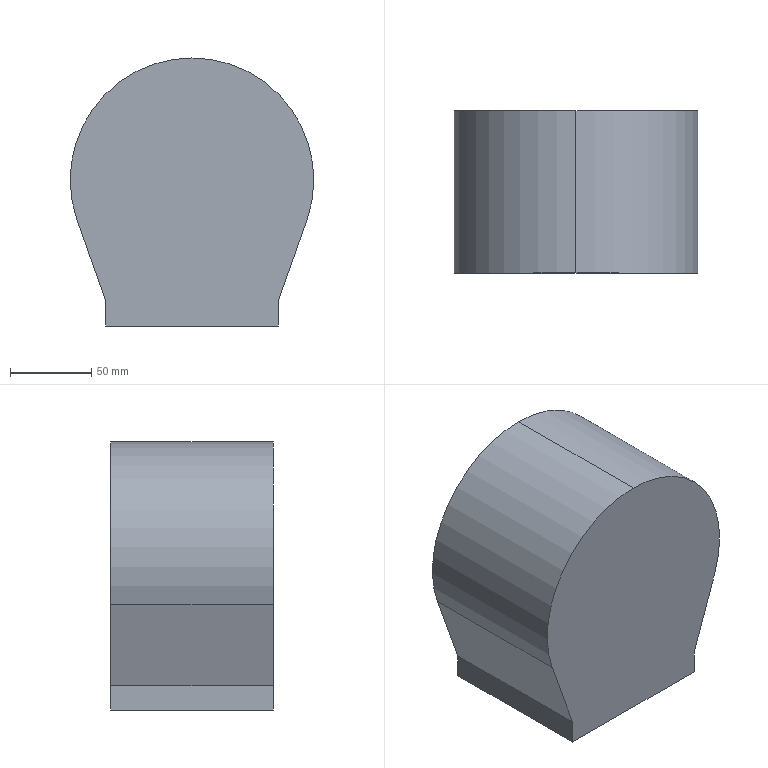Component | SolidWorks | ArmHousing-1 | 1 solid | 33 faces | box 150 x 100 x 165 mm | volume 519857 mm3 | plane 21 | cylinder 12 | commonest cylinder face diameters 4 x8 146 x2 150 x2
STEP:
#1=COLOUR_RGB('',0.7922,0.8196,0.9333);
#2=FILL_AREA_STYLE_COLOUR('',#1);
#3=FILL_AREA_STYLE('',(#2));
#4=SURFACE_STYLE_FILL_AREA(#3);
#5=SURFACE_SIDE_STYLE('',(#4));
#6=SURFACE_STYLE_USAGE(.BOTH.,#5);
#7=PRESENTATION_STYLE_ASSIGNMENT((#6));
#8=CARTESIAN_POINT('',(21.418,34.134,-80.807));
#9=VERTEX_POINT('',#8);
#10=CARTESIAN_POINT('',(21.418,34.134,-80.65));
#11=VERTEX_POINT('',#10);
#12=CARTESIAN_POINT('',(21.418,34.134,-80.729));
#13=DIRECTION('',(0.,1.,-0.));
#14=DIRECTION('',(0.,0.,1.));
#15=AXIS2_PLACEMENT_3D('',#12,#13,#14);
#16=CIRCLE('',#15,0.07874);
#17=EDGE_CURVE('',#9,#11,#16,.T.);
#18=ORIENTED_EDGE('',*,*,#17,.F.);
#19=CARTESIAN_POINT('',(21.418,34.724,-80.807));
#20=VERTEX_POINT('',#19);
#21=CARTESIAN_POINT('',(21.418,34.134,-80.807));
#22=DIRECTION('',(0.,1.,-0.));
#23=VECTOR('',#22,39.37);
#24=LINE('',#21,#23);
#25=EDGE_CURVE('',#9,#20,#24,.T.);
#26=ORIENTED_EDGE('',*,*,#25,.T.);
#27=CARTESIAN_POINT('',(21.418,34.724,-80.65));
#28=VERTEX_POINT('',#27);
#29=CARTESIAN_POINT('',(21.418,34.724,-80.729));
#30=DIRECTION('',(0.,1.,-0.));
#31=DIRECTION('',(0.,0.,1.));
#32=AXIS2_PLACEMENT_3D('',#29,#30,#31);
#33=CIRCLE('',#32,0.07874);
#34=EDGE_CURVE('',#20,#28,#33,.T.);
#35=ORIENTED_EDGE('',*,*,#34,.T.);
#36=CARTESIAN_POINT('',(21.418,34.134,-80.65));
#37=DIRECTION('',(0.,1.,-0.));
#38=VECTOR('',#37,39.37);
#39=LINE('',#36,#38);
#40=EDGE_CURVE('',#11,#28,#39,.T.);
#41=ORIENTED_EDGE('',*,*,#40,.F.);
#42=EDGE_LOOP('',(#18,#26,#35,#41));
#43=FACE_OUTER_BOUND('',#42,.T.);
#44=CARTESIAN_POINT('',(21.418,34.134,-80.729));
#45=DIRECTION('',(0.,1.,-0.));
#46=DIRECTION('',(0.,0.,1.));
#47=AXIS2_PLACEMENT_3D('',#44,#45,#46);
#48=CYLINDRICAL_SURFACE('',#47,0.07874);
#49=ADVANCED_FACE('',(#43),#48,.F.);
#50=CARTESIAN_POINT('',(24.758,34.134,-80.807));
#51=VERTEX_POINT('',#50);
#52=CARTESIAN_POINT('',(24.758,34.134,-80.65));
#53=VERTEX_POINT('',#52);
#54=CARTESIAN_POINT('',(24.758,34.134,-80.729));
#55=DIRECTION('',(0.,1.,-0.));
#56=DIRECTION('',(0.,0.,1.));
#57=AXIS2_PLACEMENT_3D('',#54,#55,#56);
#58=CIRCLE('',#57,0.07874);
#59=EDGE_CURVE('',#51,#53,#58,.T.);
#60=ORIENTED_EDGE('',*,*,#59,.F.);
#61=CARTESIAN_POINT('',(24.758,34.724,-80.807));
#62=VERTEX_POINT('',#61);
#63=CARTESIAN_POINT('',(24.758,34.134,-80.807));
#64=DIRECTION('',(0.,1.,-0.));
#65=VECTOR('',#64,39.37);
#66=LINE('',#63,#65);
#67=EDGE_CURVE('',#51,#62,#66,.T.);
#68=ORIENTED_EDGE('',*,*,#67,.T.);
#69=CARTESIAN_POINT('',(24.758,34.724,-80.65));
#70=VERTEX_POINT('',#69);
#71=CARTESIAN_POINT('',(24.758,34.724,-80.729));
#72=DIRECTION('',(0.,1.,-0.));
#73=DIRECTION('',(0.,0.,1.));
#74=AXIS2_PLACEMENT_3D('',#71,#72,#73);
#75=CIRCLE('',#74,0.07874);
#76=EDGE_CURVE('',#62,#70,#75,.T.);
#77=ORIENTED_EDGE('',*,*,#76,.T.);
#78=CARTESIAN_POINT('',(24.758,34.134,-80.65));
#79=DIRECTION('',(0.,1.,-0.));
#80=VECTOR('',#79,39.37);
#81=LINE('',#78,#80);
#82=EDGE_CURVE('',#53,#70,#81,.T.);
#83=ORIENTED_EDGE('',*,*,#82,.F.);
#84=EDGE_LOOP('',(#60,#68,#77,#83));
#85=FACE_OUTER_BOUND('',#84,.T.);
#86=CARTESIAN_POINT('',(24.758,34.134,-80.729));
#87=DIRECTION('',(0.,1.,-0.));
#88=DIRECTION('',(0.,0.,1.));
#89=AXIS2_PLACEMENT_3D('',#86,#87,#88);
#90=CYLINDRICAL_SURFACE('',#89,0.07874);
#91=ADVANCED_FACE('',(#85),#90,.F.);
#92=CARTESIAN_POINT('',(24.758,34.134,-84.148));
#93=VERTEX_POINT('',#92);
#94=CARTESIAN_POINT('',(24.758,34.134,-83.991));
#95=VERTEX_POINT('',#94);
#96=CARTESIAN_POINT('',(24.758,34.134,-84.069));
#97=DIRECTION('',(0.,1.,-0.));
#98=DIRECTION('',(0.,0.,1.));
#99=AXIS2_PLACEMENT_3D('',#96,#97,#98);
#100=CIRCLE('',#99,0.07874);
#101=EDGE_CURVE('',#93,#95,#100,.T.);
#102=ORIENTED_EDGE('',*,*,#101,.F.);
#103=CARTESIAN_POINT('',(24.758,34.724,-84.148));
#104=VERTEX_POINT('',#103);
#105=CARTESIAN_POINT('',(24.758,34.134,-84.148));
#106=DIRECTION('',(0.,1.,-0.));
#107=VECTOR('',#106,39.37);
#108=LINE('',#105,#107);
#109=EDGE_CURVE('',#93,#104,#108,.T.);
#110=ORIENTED_EDGE('',*,*,#109,.T.);
#111=CARTESIAN_POINT('',(24.758,34.724,-83.991));
#112=VERTEX_POINT('',#111);
#113=CARTESIAN_POINT('',(24.758,34.724,-84.069));
#114=DIRECTION('',(0.,1.,-0.));
#115=DIRECTION('',(0.,0.,1.));
#116=AXIS2_PLACEMENT_3D('',#113,#114,#115);
#117=CIRCLE('',#116,0.07874);
#118=EDGE_CURVE('',#104,#112,#117,.T.);
#119=ORIENTED_EDGE('',*,*,#118,.T.);
#120=CARTESIAN_POINT('',(24.758,34.134,-83.991));
#121=DIRECTION('',(0.,1.,-0.));
#122=VECTOR('',#121,39.37);
#123=LINE('',#120,#122);
#124=EDGE_CURVE('',#95,#112,#123,.T.);
#125=ORIENTED_EDGE('',*,*,#124,.F.);
#126=EDGE_LOOP('',(#102,#110,#119,#125));
#127=FACE_OUTER_BOUND('',#126,.T.);
#128=CARTESIAN_POINT('',(24.758,34.134,-84.069));
#129=DIRECTION('',(0.,1.,-0.));
#130=DIRECTION('',(0.,0.,1.));
#131=AXIS2_PLACEMENT_3D('',#128,#129,#130);
#132=CYLINDRICAL_SURFACE('',#131,0.07874);
#133=ADVANCED_FACE('',(#127),#132,.F.);
#134=CARTESIAN_POINT('',(21.418,34.134,-84.148));
#135=VERTEX_POINT('',#134);
#136=CARTESIAN_POINT('',(21.418,34.134,-83.991));
#137=VERTEX_POINT('',#136);
#138=CARTESIAN_POINT('',(21.418,34.134,-84.069));
#139=DIRECTION('',(0.,1.,-0.));
#140=DIRECTION('',(0.,0.,1.));
#141=AXIS2_PLACEMENT_3D('',#138,#139,#140);
#142=CIRCLE('',#141,0.07874);
#143=EDGE_CURVE('',#135,#137,#142,.T.);
#144=ORIENTED_EDGE('',*,*,#143,.F.);
#145=CARTESIAN_POINT('',(21.418,34.724,-84.148));
#146=VERTEX_POINT('',#145);
#147=CARTESIAN_POINT('',(21.418,34.134,-84.148));
#148=DIRECTION('',(0.,1.,-0.));
#149=VECTOR('',#148,39.37);
#150=LINE('',#147,#149);
#151=EDGE_CURVE('',#135,#146,#150,.T.);
#152=ORIENTED_EDGE('',*,*,#151,.T.);
#153=CARTESIAN_POINT('',(21.418,34.724,-83.991));
#154=VERTEX_POINT('',#153);
#155=CARTESIAN_POINT('',(21.418,34.724,-84.069));
#156=DIRECTION('',(0.,1.,-0.));
#157=DIRECTION('',(0.,0.,1.));
#158=AXIS2_PLACEMENT_3D('',#155,#156,#157);
#159=CIRCLE('',#158,0.07874);
#160=EDGE_CURVE('',#146,#154,#159,.T.);
#161=ORIENTED_EDGE('',*,*,#160,.T.);
#162=CARTESIAN_POINT('',(21.418,34.134,-83.991));
#163=DIRECTION('',(0.,1.,-0.));
#164=VECTOR('',#163,39.37);
#165=LINE('',#162,#164);
#166=EDGE_CURVE('',#137,#154,#165,.T.);
#167=ORIENTED_EDGE('',*,*,#166,.F.);
#168=EDGE_LOOP('',(#144,#152,#161,#167));
#169=FACE_OUTER_BOUND('',#168,.T.);
#170=CARTESIAN_POINT('',(21.418,34.134,-84.069));
#171=DIRECTION('',(0.,1.,-0.));
#172=DIRECTION('',(0.,0.,1.));
#173=AXIS2_PLACEMENT_3D('',#170,#171,#172);
#174=CYLINDRICAL_SURFACE('',#173,0.07874);
#175=ADVANCED_FACE('',(#169),#174,.F.);
#176=CARTESIAN_POINT('',(23.088,34.724,-79.525));
#177=VERTEX_POINT('',#176);
#178=CARTESIAN_POINT('',(25.796,34.724,-83.361));
#179=VERTEX_POINT('',#178);
#180=CARTESIAN_POINT('',(23.088,34.724,-82.399));
#181=DIRECTION('',(0.,1.,-0.));
#182=DIRECTION('',(0.,0.,1.));
#183=AXIS2_PLACEMENT_3D('',#180,#181,#182);
#184=CIRCLE('',#183,2.874);
#185=EDGE_CURVE('',#177,#179,#184,.T.);
#186=ORIENTED_EDGE('',*,*,#185,.F.);
#187=CARTESIAN_POINT('',(23.088,37.795,-79.525));
#188=VERTEX_POINT('',#187);
#189=CARTESIAN_POINT('',(23.088,25.507,-79.525));
#190=DIRECTION('',(0.,1.,-0.));
#191=VECTOR('',#190,39.37);
#192=LINE('',#189,#191);
#193=EDGE_CURVE('',#177,#188,#192,.T.);
#194=ORIENTED_EDGE('',*,*,#193,.T.);
#195=CARTESIAN_POINT('',(25.796,37.795,-83.361));
#196=VERTEX_POINT('',#195);
#197=CARTESIAN_POINT('',(23.088,37.795,-82.399));
#198=DIRECTION('',(0.,1.,-0.));
#199=DIRECTION('',(0.,0.,1.));
#200=AXIS2_PLACEMENT_3D('',#197,#198,#199);
#201=CIRCLE('',#200,2.874);
#202=EDGE_CURVE('',#188,#196,#201,.T.);
#203=ORIENTED_EDGE('',*,*,#202,.T.);
#204=CARTESIAN_POINT('',(25.796,25.507,-83.361));
#205=DIRECTION('',(0.,1.,-0.));
#206=VECTOR('',#205,39.37);
#207=LINE('',#204,#206);
#208=EDGE_CURVE('',#179,#196,#207,.T.);
#209=ORIENTED_EDGE('',*,*,#208,.F.);
#210=EDGE_LOOP('',(#186,#194,#203,#209));
#211=FACE_OUTER_BOUND('',#210,.T.);
#212=CARTESIAN_POINT('',(23.088,25.507,-82.399));
#213=DIRECTION('',(0.,1.,-0.));
#214=DIRECTION('',(0.,0.,1.));
#215=AXIS2_PLACEMENT_3D('',#212,#213,#214);
#216=CYLINDRICAL_SURFACE('',#215,2.874);
#217=ADVANCED_FACE('',(#211),#216,.F.);
#218=CARTESIAN_POINT('',(20.306,33.858,-83.387));
#219=VERTEX_POINT('',#218);
#220=CARTESIAN_POINT('',(23.088,33.858,-79.446));
#221=VERTEX_POINT('',#220);
#222=CARTESIAN_POINT('',(23.088,33.858,-82.399));
#223=DIRECTION('',(0.,1.,-0.));
#224=DIRECTION('',(0.,0.,-1.));
#225=AXIS2_PLACEMENT_3D('',#222,#223,#224);
#226=CIRCLE('',#225,2.953);
#227=EDGE_CURVE('',#219,#221,#226,.T.);
#228=ORIENTED_EDGE('',*,*,#227,.T.);
#229=CARTESIAN_POINT('',(23.088,37.795,-79.446));
#230=VERTEX_POINT('',#229);
#231=CARTESIAN_POINT('',(23.088,25.507,-79.446));
#232=DIRECTION('',(0.,1.,-0.));
#233=VECTOR('',#232,39.37);
#234=LINE('',#231,#233);
#235=EDGE_CURVE('',#221,#230,#234,.T.);
#236=ORIENTED_EDGE('',*,*,#235,.T.);
#237=CARTESIAN_POINT('',(20.306,37.795,-83.387));
#238=VERTEX_POINT('',#237);
#239=CARTESIAN_POINT('',(23.088,37.795,-82.399));
#240=DIRECTION('',(0.,1.,-0.));
#241=DIRECTION('',(0.,0.,1.));
#242=AXIS2_PLACEMENT_3D('',#239,#240,#241);
#243=CIRCLE('',#242,2.953);
#244=EDGE_CURVE('',#238,#230,#243,.T.);
#245=ORIENTED_EDGE('',*,*,#244,.F.);
#246=CARTESIAN_POINT('',(20.306,27.957,-83.387));
#247=DIRECTION('',(0.,1.,-0.));
#248=VECTOR('',#247,39.37);
#249=LINE('',#246,#248);
#250=EDGE_CURVE('',#219,#238,#249,.T.);
#251=ORIENTED_EDGE('',*,*,#250,.F.);
#252=EDGE_LOOP('',(#228,#236,#245,#251));
#253=FACE_OUTER_BOUND('',#252,.T.);
#254=CARTESIAN_POINT('',(23.088,25.507,-82.399));
#255=DIRECTION('',(0.,1.,-0.));
#256=DIRECTION('',(0.,0.,1.));
#257=AXIS2_PLACEMENT_3D('',#254,#255,#256);
#258=CYLINDRICAL_SURFACE('',#257,2.953);
#259=ADVANCED_FACE('',(#253),#258,.T.);
#260=CARTESIAN_POINT('',(21.082,37.795,-85.338));
#261=VERTEX_POINT('',#260);
#262=CARTESIAN_POINT('',(20.38,37.795,-83.361));
#263=VERTEX_POINT('',#262);
#264=CARTESIAN_POINT('',(20.335,37.795,-83.234));
#265=DIRECTION('',(-0.3347,0.,0.9423));
#266=VECTOR('',#265,39.37);
#267=LINE('',#264,#266);
#268=EDGE_CURVE('',#261,#263,#267,.T.);
#269=ORIENTED_EDGE('',*,*,#268,.F.);
#270=CARTESIAN_POINT('',(21.082,37.795,-85.864));
#271=VERTEX_POINT('',#270);
#272=CARTESIAN_POINT('',(21.082,37.795,-85.352));
#273=DIRECTION('',(-0.,-0.,-1.));
#274=VECTOR('',#273,39.37);
#275=LINE('',#272,#274);
#276=EDGE_CURVE('',#261,#271,#275,.T.);
#277=ORIENTED_EDGE('',*,*,#276,.T.);
#278=CARTESIAN_POINT('',(25.094,37.795,-85.864));
#279=VERTEX_POINT('',#278);
#280=CARTESIAN_POINT('',(14.372,37.795,-85.864));
#281=DIRECTION('',(1.,-0.,-0.));
#282=VECTOR('',#281,39.37);
#283=LINE('',#280,#282);
#284=EDGE_CURVE('',#271,#279,#283,.T.);
#285=ORIENTED_EDGE('',*,*,#284,.T.);
#286=CARTESIAN_POINT('',(25.094,37.795,-85.338));
#287=VERTEX_POINT('',#286);
#288=CARTESIAN_POINT('',(25.094,37.795,-85.352));
#289=DIRECTION('',(-0.,-0.,-1.));
#290=VECTOR('',#289,39.37);
#291=LINE('',#288,#290);
#292=EDGE_CURVE('',#287,#279,#291,.T.);
#293=ORIENTED_EDGE('',*,*,#292,.F.);
#294=CARTESIAN_POINT('',(23.888,37.795,-88.732));
#295=DIRECTION('',(0.3347,0.,0.9423));
#296=VECTOR('',#295,39.37);
#297=LINE('',#294,#296);
#298=EDGE_CURVE('',#287,#196,#297,.T.);
#299=ORIENTED_EDGE('',*,*,#298,.T.);
#300=ORIENTED_EDGE('',*,*,#202,.F.);
#301=CARTESIAN_POINT('',(23.088,37.795,-82.399));
#302=DIRECTION('',(0.,1.,-0.));
#303=DIRECTION('',(0.,0.,1.));
#304=AXIS2_PLACEMENT_3D('',#301,#302,#303);
#305=CIRCLE('',#304,2.874);
#306=EDGE_CURVE('',#263,#188,#305,.T.);
#307=ORIENTED_EDGE('',*,*,#306,.F.);
#308=EDGE_LOOP('',(#269,#277,#285,#293,#299,#300,#307));
#309=FACE_BOUND('',#308,.T.);
#310=CARTESIAN_POINT('',(21.003,37.795,-85.352));
#311=VERTEX_POINT('',#310);
#312=CARTESIAN_POINT('',(20.447,37.795,-83.784));
#313=DIRECTION('',(-0.3347,0.,0.9423));
#314=VECTOR('',#313,39.37);
#315=LINE('',#312,#314);
#316=EDGE_CURVE('',#311,#238,#315,.T.);
#317=ORIENTED_EDGE('',*,*,#316,.T.);
#318=ORIENTED_EDGE('',*,*,#244,.T.);
#319=CARTESIAN_POINT('',(25.871,37.795,-83.387));
#320=VERTEX_POINT('',#319);
#321=CARTESIAN_POINT('',(23.088,37.795,-82.399));
#322=DIRECTION('',(0.,1.,-0.));
#323=DIRECTION('',(0.,0.,1.));
#324=AXIS2_PLACEMENT_3D('',#321,#322,#323);
#325=CIRCLE('',#324,2.953);
#326=EDGE_CURVE('',#230,#320,#325,.T.);
#327=ORIENTED_EDGE('',*,*,#326,.T.);
#328=CARTESIAN_POINT('',(25.173,37.795,-85.352));
#329=VERTEX_POINT('',#328);
#330=CARTESIAN_POINT('',(23.776,37.795,-89.283));
#331=DIRECTION('',(0.3347,0.,0.9423));
#332=VECTOR('',#331,39.37);
#333=LINE('',#330,#332);
#334=EDGE_CURVE('',#329,#320,#333,.T.);
#335=ORIENTED_EDGE('',*,*,#334,.F.);
#336=CARTESIAN_POINT('',(25.173,37.795,-85.942));
#337=VERTEX_POINT('',#336);
#338=CARTESIAN_POINT('',(25.173,37.795,-85.352));
#339=DIRECTION('',(-0.,-0.,-1.));
#340=VECTOR('',#339,39.37);
#341=LINE('',#338,#340);
#342=EDGE_CURVE('',#329,#337,#341,.T.);
#343=ORIENTED_EDGE('',*,*,#342,.T.);
#344=CARTESIAN_POINT('',(21.003,37.795,-85.942));
#345=VERTEX_POINT('',#344);
#346=CARTESIAN_POINT('',(14.372,37.795,-85.942));
#347=DIRECTION('',(1.,-0.,-0.));
#348=VECTOR('',#347,39.37);
#349=LINE('',#346,#348);
#350=EDGE_CURVE('',#345,#337,#349,.T.);
#351=ORIENTED_EDGE('',*,*,#350,.F.);
#352=CARTESIAN_POINT('',(21.003,37.795,-85.352));
#353=DIRECTION('',(-0.,-0.,-1.));
#354=VECTOR('',#353,39.37);
#355=LINE('',#352,#354);
#356=EDGE_CURVE('',#311,#345,#355,.T.);
#357=ORIENTED_EDGE('',*,*,#356,.F.);
#358=EDGE_LOOP('',(#317,#318,#327,#335,#343,#351,#357));
#359=FACE_OUTER_BOUND('',#358,.T.);
#360=CARTESIAN_POINT('',(14.372,37.795,-85.352));
#361=DIRECTION('',(0.,1.,-0.));
#362=DIRECTION('',(0.,0.,1.));
#363=AXIS2_PLACEMENT_3D('',#360,#361,#362);
#364=PLANE('',#363);
#365=ADVANCED_FACE('',(#309,#359),#364,.T.);
#366=CARTESIAN_POINT('',(21.003,33.858,-85.942));
#367=VERTEX_POINT('',#366);
#368=CARTESIAN_POINT('',(21.003,55.591,-85.942));
#369=DIRECTION('',(-0.,-1.,0.));
#370=VECTOR('',#369,39.37);
#371=LINE('',#368,#370);
#372=EDGE_CURVE('',#345,#367,#371,.T.);
#373=ORIENTED_EDGE('',*,*,#372,.T.);
#374=CARTESIAN_POINT('',(21.003,33.858,-85.352));
#375=VERTEX_POINT('',#374);
#376=CARTESIAN_POINT('',(21.003,33.858,-85.352));
#377=DIRECTION('',(-0.,-0.,-1.));
#378=VECTOR('',#377,39.37);
#379=LINE('',#376,#378);
#380=EDGE_CURVE('',#375,#367,#379,.T.);
#381=ORIENTED_EDGE('',*,*,#380,.F.);
#382=CARTESIAN_POINT('',(21.003,55.591,-85.352));
#383=DIRECTION('',(-0.,-1.,0.));
#384=VECTOR('',#383,39.37);
#385=LINE('',#382,#384);
#386=EDGE_CURVE('',#311,#375,#385,.T.);
#387=ORIENTED_EDGE('',*,*,#386,.F.);
#388=ORIENTED_EDGE('',*,*,#356,.T.);
#389=EDGE_LOOP('',(#373,#381,#387,#388));
#390=FACE_OUTER_BOUND('',#389,.T.);
#391=CARTESIAN_POINT('',(21.003,55.591,-85.352));
#392=DIRECTION('',(1.,-0.,-0.));
#393=DIRECTION('',(0.,1.,-0.));
#394=AXIS2_PLACEMENT_3D('',#391,#392,#393);
#395=PLANE('',#394);
#396=ADVANCED_FACE('',(#390),#395,.F.);
#397=CARTESIAN_POINT('',(25.173,33.858,-85.352));
#398=VERTEX_POINT('',#397);
#399=CARTESIAN_POINT('',(25.871,33.858,-83.387));
#400=VERTEX_POINT('',#399);
#401=CARTESIAN_POINT('',(23.776,33.858,-89.283));
#402=DIRECTION('',(0.3347,0.,0.9423));
#403=VECTOR('',#402,39.37);
#404=LINE('',#401,#403);
#405=EDGE_CURVE('',#398,#400,#404,.T.);
#406=ORIENTED_EDGE('',*,*,#405,.T.);
#407=CARTESIAN_POINT('',(23.088,33.858,-82.399));
#408=DIRECTION('',(0.,1.,-0.));
#409=DIRECTION('',(0.,0.,-1.));
#410=AXIS2_PLACEMENT_3D('',#407,#408,#409);
#411=CIRCLE('',#410,2.953);
#412=EDGE_CURVE('',#221,#400,#411,.T.);
#413=ORIENTED_EDGE('',*,*,#412,.F.);
#414=ORIENTED_EDGE('',*,*,#227,.F.);
#415=CARTESIAN_POINT('',(20.447,33.858,-83.784));
#416=DIRECTION('',(-0.3347,0.,0.9423));
#417=VECTOR('',#416,39.37);
#418=LINE('',#415,#417);
#419=EDGE_CURVE('',#375,#219,#418,.T.);
#420=ORIENTED_EDGE('',*,*,#419,.F.);
#421=ORIENTED_EDGE('',*,*,#380,.T.);
#422=CARTESIAN_POINT('',(25.173,33.858,-85.942));
#423=VERTEX_POINT('',#422);
#424=CARTESIAN_POINT('',(14.372,33.858,-85.942));
#425=DIRECTION('',(-1.,0.,0.));
#426=VECTOR('',#425,39.37);
#427=LINE('',#424,#426);
#428=EDGE_CURVE('',#423,#367,#427,.T.);
#429=ORIENTED_EDGE('',*,*,#428,.F.);
#430=CARTESIAN_POINT('',(25.173,33.858,-85.352));
#431=DIRECTION('',(-0.,-0.,-1.));
#432=VECTOR('',#431,39.37);
#433=LINE('',#430,#432);
#434=EDGE_CURVE('',#398,#423,#433,.T.);
#435=ORIENTED_EDGE('',*,*,#434,.F.);
#436=EDGE_LOOP('',(#406,#413,#414,#420,#421,#429,#435));
#437=FACE_OUTER_BOUND('',#436,.T.);
#438=CARTESIAN_POINT('',(14.372,33.858,-85.352));
#439=DIRECTION('',(0.,-1.,0.));
#440=DIRECTION('',(-0.,-0.,-1.));
#441=AXIS2_PLACEMENT_3D('',#438,#439,#440);
#442=PLANE('',#441);
#443=ADVANCED_FACE('',(#437),#442,.T.);
#444=CARTESIAN_POINT('',(25.173,55.591,-85.942));
#445=DIRECTION('',(0.,1.,-0.));
#446=VECTOR('',#445,39.37);
#447=LINE('',#444,#446);
#448=EDGE_CURVE('',#423,#337,#447,.T.);
#449=ORIENTED_EDGE('',*,*,#448,.T.);
#450=ORIENTED_EDGE('',*,*,#342,.F.);
#451=CARTESIAN_POINT('',(25.173,55.591,-85.352));
#452=DIRECTION('',(0.,1.,-0.));
#453=VECTOR('',#452,39.37);
#454=LINE('',#451,#453);
#455=EDGE_CURVE('',#398,#329,#454,.T.);
#456=ORIENTED_EDGE('',*,*,#455,.F.);
#457=ORIENTED_EDGE('',*,*,#434,.T.);
#458=EDGE_LOOP('',(#449,#450,#456,#457));
#459=FACE_OUTER_BOUND('',#458,.T.);
#460=CARTESIAN_POINT('',(25.173,55.591,-85.352));
#461=DIRECTION('',(-1.,0.,0.));
#462=DIRECTION('',(-0.,-0.,-1.));
#463=AXIS2_PLACEMENT_3D('',#460,#461,#462);
#464=PLANE('',#463);
#465=ADVANCED_FACE('',(#459),#464,.F.);
#466=CARTESIAN_POINT('',(21.978,37.075,-85.942));
#467=VERTEX_POINT('',#466);
#468=CARTESIAN_POINT('',(21.978,34.764,-85.942));
#469=VERTEX_POINT('',#468);
#470=CARTESIAN_POINT('',(21.978,55.591,-85.942));
#471=DIRECTION('',(0.,-1.,0.));
#472=VECTOR('',#471,39.37);
#473=LINE('',#470,#472);
#474=EDGE_CURVE('',#467,#469,#473,.T.);
#475=ORIENTED_EDGE('',*,*,#474,.T.);
#476=CARTESIAN_POINT('',(24.34,34.764,-85.942));
#477=VERTEX_POINT('',#476);
#478=CARTESIAN_POINT('',(24.34,34.764,-85.942));
#479=DIRECTION('',(-1.,0.,0.));
#480=VECTOR('',#479,39.37);
#481=LINE('',#478,#480);
#482=EDGE_CURVE('',#477,#469,#481,.T.);
#483=ORIENTED_EDGE('',*,*,#482,.F.);
#484=CARTESIAN_POINT('',(24.34,37.075,-85.942));
#485=VERTEX_POINT('',#484);
#486=CARTESIAN_POINT('',(24.34,55.591,-85.942));
#487=DIRECTION('',(0.,1.,-0.));
#488=VECTOR('',#487,39.37);
#489=LINE('',#486,#488);
#490=EDGE_CURVE('',#477,#485,#489,.T.);
#491=ORIENTED_EDGE('',*,*,#490,.T.);
#492=CARTESIAN_POINT('',(14.372,37.075,-85.942));
#493=DIRECTION('',(-1.,-0.,0.));
#494=VECTOR('',#493,39.37);
#495=LINE('',#492,#494);
#496=EDGE_CURVE('',#485,#467,#495,.T.);
#497=ORIENTED_EDGE('',*,*,#496,.T.);
#498=EDGE_LOOP('',(#475,#483,#491,#497));
#499=FACE_BOUND('',#498,.T.);
#500=ORIENTED_EDGE('',*,*,#350,.T.);
#501=ORIENTED_EDGE('',*,*,#448,.F.);
#502=ORIENTED_EDGE('',*,*,#428,.T.);
#503=ORIENTED_EDGE('',*,*,#372,.F.);
#504=EDGE_LOOP('',(#500,#501,#502,#503));
#505=FACE_OUTER_BOUND('',#504,.T.);
#506=CARTESIAN_POINT('',(14.372,55.591,-85.942));
#507=DIRECTION('',(0.,0.,1.));
#508=DIRECTION('',(0.,-1.,0.));
#509=AXIS2_PLACEMENT_3D('',#506,#507,#508);
#510=PLANE('',#509);
#511=ADVANCED_FACE('',(#499,#505),#510,.F.);
#512=ORIENTED_EDGE('',*,*,#405,.F.);
#513=ORIENTED_EDGE('',*,*,#455,.T.);
#514=ORIENTED_EDGE('',*,*,#334,.T.);
#515=CARTESIAN_POINT('',(25.871,27.957,-83.387));
#516=DIRECTION('',(0.,1.,-0.));
#517=VECTOR('',#516,39.37);
#518=LINE('',#515,#517);
#519=EDGE_CURVE('',#400,#320,#518,.T.);
#520=ORIENTED_EDGE('',*,*,#519,.F.);
#521=EDGE_LOOP('',(#512,#513,#514,#520));
#522=FACE_OUTER_BOUND('',#521,.T.);
#523=CARTESIAN_POINT('',(23.776,27.957,-89.283));
#524=DIRECTION('',(-0.9423,0.,0.3347));
#525=DIRECTION('',(-0.3347,-0.,-0.9423));
#526=AXIS2_PLACEMENT_3D('',#523,#524,#525);
#527=PLANE('',#526);
#528=ADVANCED_FACE('',(#522),#527,.F.);
#529=ORIENTED_EDGE('',*,*,#386,.T.);
#530=ORIENTED_EDGE('',*,*,#419,.T.);
#531=ORIENTED_EDGE('',*,*,#250,.T.);
#532=ORIENTED_EDGE('',*,*,#316,.F.);
#533=EDGE_LOOP('',(#529,#530,#531,#532));
#534=FACE_OUTER_BOUND('',#533,.T.);
#535=CARTESIAN_POINT('',(20.447,27.957,-83.784));
#536=DIRECTION('',(-0.9423,-0.,-0.3347));
#537=DIRECTION('',(0.3347,-0.,-0.9423));
#538=AXIS2_PLACEMENT_3D('',#535,#536,#537);
#539=PLANE('',#538);
#540=ADVANCED_FACE('',(#534),#539,.T.);
#541=ORIENTED_EDGE('',*,*,#235,.F.);
#542=ORIENTED_EDGE('',*,*,#412,.T.);
#543=ORIENTED_EDGE('',*,*,#519,.T.);
#544=ORIENTED_EDGE('',*,*,#326,.F.);
#545=EDGE_LOOP('',(#541,#542,#543,#544));
#546=FACE_OUTER_BOUND('',#545,.T.);
#547=CARTESIAN_POINT('',(23.088,25.507,-82.399));
#548=DIRECTION('',(0.,1.,-0.));
#549=DIRECTION('',(0.,0.,1.));
#550=AXIS2_PLACEMENT_3D('',#547,#548,#549);
#551=CYLINDRICAL_SURFACE('',#550,2.953);
#552=ADVANCED_FACE('',(#546),#551,.T.);
#553=CARTESIAN_POINT('',(21.082,34.724,-85.864));
#554=VERTEX_POINT('',#553);
#555=CARTESIAN_POINT('',(21.082,34.724,-85.338));
#556=VERTEX_POINT('',#555);
#557=CARTESIAN_POINT('',(21.082,34.724,-85.864));
#558=DIRECTION('',(0.,0.,1.));
#559=VECTOR('',#558,39.37);
#560=LINE('',#557,#559);
#561=EDGE_CURVE('',#554,#556,#560,.T.);
#562=ORIENTED_EDGE('',*,*,#561,.F.);
#563=CARTESIAN_POINT('',(21.082,55.591,-85.864));
#564=DIRECTION('',(-0.,-1.,0.));
#565=VECTOR('',#564,39.37);
#566=LINE('',#563,#565);
#567=EDGE_CURVE('',#271,#554,#566,.T.);
#568=ORIENTED_EDGE('',*,*,#567,.F.);
#569=ORIENTED_EDGE('',*,*,#276,.F.);
#570=CARTESIAN_POINT('',(21.082,27.957,-85.338));
#571=DIRECTION('',(-0.,-1.,0.));
#572=VECTOR('',#571,39.37);
#573=LINE('',#570,#572);
#574=EDGE_CURVE('',#261,#556,#573,.T.);
#575=ORIENTED_EDGE('',*,*,#574,.T.);
#576=EDGE_LOOP('',(#562,#568,#569,#575));
#577=FACE_OUTER_BOUND('',#576,.T.);
#578=CARTESIAN_POINT('',(21.082,55.591,-85.352));
#579=DIRECTION('',(1.,-0.,-0.));
#580=DIRECTION('',(0.,1.,-0.));
#581=AXIS2_PLACEMENT_3D('',#578,#579,#580);
#582=PLANE('',#581);
#583=ADVANCED_FACE('',(#577),#582,.T.);
#584=CARTESIAN_POINT('',(25.094,34.724,-85.338));
#585=VERTEX_POINT('',#584);
#586=CARTESIAN_POINT('',(25.094,34.724,-85.864));
#587=VERTEX_POINT('',#586);
#588=CARTESIAN_POINT('',(25.094,34.724,-85.338));
#589=DIRECTION('',(-0.,-0.,-1.));
#590=VECTOR('',#589,39.37);
#591=LINE('',#588,#590);
#592=EDGE_CURVE('',#585,#587,#591,.T.);
#593=ORIENTED_EDGE('',*,*,#592,.F.);
#594=CARTESIAN_POINT('',(25.094,55.591,-85.338));
#595=DIRECTION('',(0.,1.,-0.));
#596=VECTOR('',#595,39.37);
#597=LINE('',#594,#596);
#598=EDGE_CURVE('',#585,#287,#597,.T.);
#599=ORIENTED_EDGE('',*,*,#598,.T.);
#600=ORIENTED_EDGE('',*,*,#292,.T.);
#601=CARTESIAN_POINT('',(25.094,55.591,-85.864));
#602=DIRECTION('',(0.,1.,-0.));
#603=VECTOR('',#602,39.37);
#604=LINE('',#601,#603);
#605=EDGE_CURVE('',#587,#279,#604,.T.);
#606=ORIENTED_EDGE('',*,*,#605,.F.);
#607=EDGE_LOOP('',(#593,#599,#600,#606));
#608=FACE_OUTER_BOUND('',#607,.T.);
#609=CARTESIAN_POINT('',(25.094,55.591,-85.352));
#610=DIRECTION('',(-1.,0.,0.));
#611=DIRECTION('',(-0.,-0.,-1.));
#612=AXIS2_PLACEMENT_3D('',#609,#610,#611);
#613=PLANE('',#612);
#614=ADVANCED_FACE('',(#608),#613,.T.);
#615=CARTESIAN_POINT('',(21.978,34.764,-85.864));
#616=VERTEX_POINT('',#615);
#617=CARTESIAN_POINT('',(24.34,34.764,-85.864));
#618=VERTEX_POINT('',#617);
#619=CARTESIAN_POINT('',(14.372,34.764,-85.864));
#620=DIRECTION('',(1.,-0.,-0.));
#621=VECTOR('',#620,39.37);
#622=LINE('',#619,#621);
#623=EDGE_CURVE('',#616,#618,#622,.T.);
#624=ORIENTED_EDGE('',*,*,#623,.F.);
#625=CARTESIAN_POINT('',(21.978,37.075,-85.864));
#626=VERTEX_POINT('',#625);
#627=CARTESIAN_POINT('',(21.978,37.075,-85.864));
#628=DIRECTION('',(0.,-1.,0.));
#629=VECTOR('',#628,39.37);
#630=LINE('',#627,#629);
#631=EDGE_CURVE('',#626,#616,#630,.T.);
#632=ORIENTED_EDGE('',*,*,#631,.F.);
#633=CARTESIAN_POINT('',(24.34,37.075,-85.864));
#634=VERTEX_POINT('',#633);
#635=CARTESIAN_POINT('',(21.978,37.075,-85.864));
#636=DIRECTION('',(-1.,-0.,0.));
#637=VECTOR('',#636,39.37);
#638=LINE('',#635,#637);
#639=EDGE_CURVE('',#634,#626,#638,.T.);
#640=ORIENTED_EDGE('',*,*,#639,.F.);
#641=CARTESIAN_POINT('',(24.34,37.075,-85.864));
#642=DIRECTION('',(0.,1.,-0.));
#643=VECTOR('',#642,39.37);
#644=LINE('',#641,#643);
#645=EDGE_CURVE('',#618,#634,#644,.T.);
#646=ORIENTED_EDGE('',*,*,#645,.F.);
#647=EDGE_LOOP('',(#624,#632,#640,#646));
#648=FACE_BOUND('',#647,.T.);
#649=CARTESIAN_POINT('',(25.094,34.724,-85.864));
#650=DIRECTION('',(-1.,0.,0.));
#651=VECTOR('',#650,39.37);
#652=LINE('',#649,#651);
#653=EDGE_CURVE('',#587,#554,#652,.T.);
#654=ORIENTED_EDGE('',*,*,#653,.F.);
#655=ORIENTED_EDGE('',*,*,#605,.T.);
#656=ORIENTED_EDGE('',*,*,#284,.F.);
#657=ORIENTED_EDGE('',*,*,#567,.T.);
#658=EDGE_LOOP('',(#654,#655,#656,#657));
#659=FACE_OUTER_BOUND('',#658,.T.);
#660=CARTESIAN_POINT('',(14.372,55.591,-85.864));
#661=DIRECTION('',(0.,0.,1.));
#662=DIRECTION('',(0.,-1.,0.));
#663=AXIS2_PLACEMENT_3D('',#660,#661,#662);
#664=PLANE('',#663);
#665=ADVANCED_FACE('',(#648,#659),#664,.T.);
#666=CARTESIAN_POINT('',(25.796,34.724,-83.361));
#667=DIRECTION('',(-0.3347,-0.,-0.9423));
#668=VECTOR('',#667,39.37);
#669=LINE('',#666,#668);
#670=EDGE_CURVE('',#179,#585,#669,.T.);
#671=ORIENTED_EDGE('',*,*,#670,.F.);
#672=ORIENTED_EDGE('',*,*,#208,.T.);
#673=ORIENTED_EDGE('',*,*,#298,.F.);
#674=ORIENTED_EDGE('',*,*,#598,.F.);
#675=EDGE_LOOP('',(#671,#672,#673,#674));
#676=FACE_OUTER_BOUND('',#675,.T.);
#677=CARTESIAN_POINT('',(23.702,27.957,-89.257));
#678=DIRECTION('',(-0.9423,0.,0.3347));
#679=DIRECTION('',(-0.3347,-0.,-0.9423));
#680=AXIS2_PLACEMENT_3D('',#677,#678,#679);
#681=PLANE('',#680);
#682=ADVANCED_FACE('',(#676),#681,.T.);
#683=CARTESIAN_POINT('',(20.38,34.724,-83.361));
#684=VERTEX_POINT('',#683);
#685=CARTESIAN_POINT('',(20.38,27.957,-83.361));
#686=DIRECTION('',(0.,1.,-0.));
#687=VECTOR('',#686,39.37);
#688=LINE('',#685,#687);
#689=EDGE_CURVE('',#684,#263,#688,.T.);
#690=ORIENTED_EDGE('',*,*,#689,.F.);
#691=CARTESIAN_POINT('',(21.082,34.724,-85.338));
#692=DIRECTION('',(-0.3347,0.,0.9423));
#693=VECTOR('',#692,39.37);
#694=LINE('',#691,#693);
#695=EDGE_CURVE('',#556,#684,#694,.T.);
#696=ORIENTED_EDGE('',*,*,#695,.F.);
#697=ORIENTED_EDGE('',*,*,#574,.F.);
#698=ORIENTED_EDGE('',*,*,#268,.T.);
#699=EDGE_LOOP('',(#690,#696,#697,#698));
#700=FACE_OUTER_BOUND('',#699,.T.);
#701=CARTESIAN_POINT('',(20.521,27.957,-83.758));
#702=DIRECTION('',(-0.9423,-0.,-0.3347));
#703=DIRECTION('',(0.3347,-0.,-0.9423));
#704=AXIS2_PLACEMENT_3D('',#701,#702,#703);
#705=PLANE('',#704);
#706=ADVANCED_FACE('',(#700),#705,.F.);
#707=ORIENTED_EDGE('',*,*,#193,.F.);
#708=CARTESIAN_POINT('',(23.088,34.724,-82.399));
#709=DIRECTION('',(0.,1.,-0.));
#710=DIRECTION('',(0.,0.,1.));
#711=AXIS2_PLACEMENT_3D('',#708,#709,#710);
#712=CIRCLE('',#711,2.874);
#713=EDGE_CURVE('',#684,#177,#712,.T.);
#714=ORIENTED_EDGE('',*,*,#713,.F.);
#715=ORIENTED_EDGE('',*,*,#689,.T.);
#716=ORIENTED_EDGE('',*,*,#306,.T.);
#717=EDGE_LOOP('',(#707,#714,#715,#716));
#718=FACE_OUTER_BOUND('',#717,.T.);
#719=CARTESIAN_POINT('',(23.088,25.507,-82.399));
#720=DIRECTION('',(0.,1.,-0.));
#721=DIRECTION('',(0.,0.,1.));
#722=AXIS2_PLACEMENT_3D('',#719,#720,#721);
#723=CYLINDRICAL_SURFACE('',#722,2.874);
#724=ADVANCED_FACE('',(#718),#723,.F.);
#725=CARTESIAN_POINT('',(21.418,34.724,-80.729));
#726=DIRECTION('',(0.,1.,-0.));
#727=DIRECTION('',(0.,0.,1.));
#728=AXIS2_PLACEMENT_3D('',#725,#726,#727);
#729=CIRCLE('',#728,0.07874);
#730=EDGE_CURVE('',#28,#20,#729,.T.);
#731=ORIENTED_EDGE('',*,*,#730,.F.);
#732=ORIENTED_EDGE('',*,*,#34,.F.);
#733=EDGE_LOOP('',(#731,#732));
#734=FACE_BOUND('',#733,.T.);
#735=CARTESIAN_POINT('',(24.758,34.724,-80.729));
#736=DIRECTION('',(0.,1.,-0.));
#737=DIRECTION('',(0.,0.,1.));
#738=AXIS2_PLACEMENT_3D('',#735,#736,#737);
#739=CIRCLE('',#738,0.07874);
#740=EDGE_CURVE('',#70,#62,#739,.T.);
#741=ORIENTED_EDGE('',*,*,#740,.F.);
#742=ORIENTED_EDGE('',*,*,#76,.F.);
#743=EDGE_LOOP('',(#741,#742));
#744=FACE_BOUND('',#743,.T.);
#745=CARTESIAN_POINT('',(24.758,34.724,-84.069));
#746=DIRECTION('',(0.,1.,-0.));
#747=DIRECTION('',(0.,0.,1.));
#748=AXIS2_PLACEMENT_3D('',#745,#746,#747);
#749=CIRCLE('',#748,0.07874);
#750=EDGE_CURVE('',#112,#104,#749,.T.);
#751=ORIENTED_EDGE('',*,*,#750,.F.);
#752=ORIENTED_EDGE('',*,*,#118,.F.);
#753=EDGE_LOOP('',(#751,#752));
#754=FACE_BOUND('',#753,.T.);
#755=CARTESIAN_POINT('',(21.418,34.724,-84.069));
#756=DIRECTION('',(0.,1.,-0.));
#757=DIRECTION('',(0.,0.,1.));
#758=AXIS2_PLACEMENT_3D('',#755,#756,#757);
#759=CIRCLE('',#758,0.07874);
#760=EDGE_CURVE('',#154,#146,#759,.T.);
#761=ORIENTED_EDGE('',*,*,#760,.F.);
#762=ORIENTED_EDGE('',*,*,#160,.F.);
#763=EDGE_LOOP('',(#761,#762));
#764=FACE_BOUND('',#763,.T.);
#765=ORIENTED_EDGE('',*,*,#713,.T.);
#766=ORIENTED_EDGE('',*,*,#185,.T.);
#767=ORIENTED_EDGE('',*,*,#670,.T.);
#768=ORIENTED_EDGE('',*,*,#592,.T.);
#769=ORIENTED_EDGE('',*,*,#653,.T.);
#770=ORIENTED_EDGE('',*,*,#561,.T.);
#771=ORIENTED_EDGE('',*,*,#695,.T.);
#772=EDGE_LOOP('',(#765,#766,#767,#768,#769,#770,#771));
#773=FACE_OUTER_BOUND('',#772,.T.);
#774=CARTESIAN_POINT('',(23.088,34.724,-82.399));
#775=DIRECTION('',(0.,1.,-0.));
#776=DIRECTION('',(0.,0.,1.));
#777=AXIS2_PLACEMENT_3D('',#774,#775,#776);
#778=PLANE('',#777);
#779=ADVANCED_FACE('',(#734,#744,#754,#764,#773),#778,.T.);
#780=CARTESIAN_POINT('',(24.34,37.075,-86.651));
#781=DIRECTION('',(0.,0.,1.));
#782=VECTOR('',#781,39.37);
#783=LINE('',#780,#782);
#784=EDGE_CURVE('',#485,#634,#783,.T.);
#785=ORIENTED_EDGE('',*,*,#784,.T.);
#786=ORIENTED_EDGE('',*,*,#639,.T.);
#787=CARTESIAN_POINT('',(21.978,37.075,-86.651));
#788=DIRECTION('',(0.,0.,1.));
#789=VECTOR('',#788,39.37);
#790=LINE('',#787,#789);
#791=EDGE_CURVE('',#467,#626,#790,.T.);
#792=ORIENTED_EDGE('',*,*,#791,.F.);
#793=ORIENTED_EDGE('',*,*,#496,.F.);
#794=EDGE_LOOP('',(#785,#786,#792,#793));
#795=FACE_OUTER_BOUND('',#794,.T.);
#796=CARTESIAN_POINT('',(21.978,37.075,-86.651));
#797=DIRECTION('',(-0.,1.,-0.));
#798=DIRECTION('',(-1.,-0.,0.));
#799=AXIS2_PLACEMENT_3D('',#796,#797,#798);
#800=PLANE('',#799);
#801=ADVANCED_FACE('',(#795),#800,.F.);
#802=ORIENTED_EDGE('',*,*,#490,.F.);
#803=CARTESIAN_POINT('',(24.34,34.764,-85.549));
#804=DIRECTION('',(-0.,-0.,-1.));
#805=VECTOR('',#804,39.37);
#806=LINE('',#803,#805);
#807=EDGE_CURVE('',#618,#477,#806,.T.);
#808=ORIENTED_EDGE('',*,*,#807,.F.);
#809=ORIENTED_EDGE('',*,*,#645,.T.);
#810=ORIENTED_EDGE('',*,*,#784,.F.);
#811=EDGE_LOOP('',(#802,#808,#809,#810));
#812=FACE_OUTER_BOUND('',#811,.T.);
#813=CARTESIAN_POINT('',(24.34,37.075,-86.651));
#814=DIRECTION('',(1.,-0.,-0.));
#815=DIRECTION('',(0.,0.,1.));
#816=AXIS2_PLACEMENT_3D('',#813,#814,#815);
#817=PLANE('',#816);
#818=ADVANCED_FACE('',(#812),#817,.F.);
#819=ORIENTED_EDGE('',*,*,#791,.T.);
#820=ORIENTED_EDGE('',*,*,#631,.T.);
#821=CARTESIAN_POINT('',(21.978,34.764,-85.549));
#822=DIRECTION('',(-0.,-0.,-1.));
#823=VECTOR('',#822,39.37);
#824=LINE('',#821,#823);
#825=EDGE_CURVE('',#616,#469,#824,.T.);
#826=ORIENTED_EDGE('',*,*,#825,.T.);
#827=ORIENTED_EDGE('',*,*,#474,.F.);
#828=EDGE_LOOP('',(#819,#820,#826,#827));
#829=FACE_OUTER_BOUND('',#828,.T.);
#830=CARTESIAN_POINT('',(21.978,37.075,-86.651));
#831=DIRECTION('',(-1.,0.,0.));
#832=DIRECTION('',(-0.,-0.,-1.));
#833=AXIS2_PLACEMENT_3D('',#830,#831,#832);
#834=PLANE('',#833);
#835=ADVANCED_FACE('',(#829),#834,.F.);
#836=ORIENTED_EDGE('',*,*,#151,.F.);
#837=CARTESIAN_POINT('',(21.418,34.134,-84.069));
#838=DIRECTION('',(0.,1.,-0.));
#839=DIRECTION('',(0.,0.,1.));
#840=AXIS2_PLACEMENT_3D('',#837,#838,#839);
#841=CIRCLE('',#840,0.07874);
#842=EDGE_CURVE('',#137,#135,#841,.T.);
#843=ORIENTED_EDGE('',*,*,#842,.F.);
#844=ORIENTED_EDGE('',*,*,#166,.T.);
#845=ORIENTED_EDGE('',*,*,#760,.T.);
#846=EDGE_LOOP('',(#836,#843,#844,#845));
#847=FACE_OUTER_BOUND('',#846,.T.);
#848=CARTESIAN_POINT('',(21.418,34.134,-84.069));
#849=DIRECTION('',(0.,1.,-0.));
#850=DIRECTION('',(0.,0.,1.));
#851=AXIS2_PLACEMENT_3D('',#848,#849,#850);
#852=CYLINDRICAL_SURFACE('',#851,0.07874);
#853=ADVANCED_FACE('',(#847),#852,.F.);
#854=ORIENTED_EDGE('',*,*,#842,.T.);
#855=ORIENTED_EDGE('',*,*,#143,.T.);
#856=EDGE_LOOP('',(#854,#855));
#857=FACE_OUTER_BOUND('',#856,.T.);
#858=CARTESIAN_POINT('',(21.418,34.134,-84.069));
#859=DIRECTION('',(0.,1.,-0.));
#860=DIRECTION('',(0.,0.,1.));
#861=AXIS2_PLACEMENT_3D('',#858,#859,#860);
#862=PLANE('',#861);
#863=ADVANCED_FACE('',(#857),#862,.T.);
#864=ORIENTED_EDGE('',*,*,#109,.F.);
#865=CARTESIAN_POINT('',(24.758,34.134,-84.069));
#866=DIRECTION('',(0.,1.,-0.));
#867=DIRECTION('',(0.,0.,1.));
#868=AXIS2_PLACEMENT_3D('',#865,#866,#867);
#869=CIRCLE('',#868,0.07874);
#870=EDGE_CURVE('',#95,#93,#869,.T.);
#871=ORIENTED_EDGE('',*,*,#870,.F.);
#872=ORIENTED_EDGE('',*,*,#124,.T.);
#873=ORIENTED_EDGE('',*,*,#750,.T.);
#874=EDGE_LOOP('',(#864,#871,#872,#873));
#875=FACE_OUTER_BOUND('',#874,.T.);
#876=CARTESIAN_POINT('',(24.758,34.134,-84.069));
#877=DIRECTION('',(0.,1.,-0.));
#878=DIRECTION('',(0.,0.,1.));
#879=AXIS2_PLACEMENT_3D('',#876,#877,#878);
#880=CYLINDRICAL_SURFACE('',#879,0.07874);
#881=ADVANCED_FACE('',(#875),#880,.F.);
#882=ORIENTED_EDGE('',*,*,#870,.T.);
#883=ORIENTED_EDGE('',*,*,#101,.T.);
#884=EDGE_LOOP('',(#882,#883));
#885=FACE_OUTER_BOUND('',#884,.T.);
#886=CARTESIAN_POINT('',(24.758,34.134,-84.069));
#887=DIRECTION('',(0.,1.,-0.));
#888=DIRECTION('',(0.,0.,1.));
#889=AXIS2_PLACEMENT_3D('',#886,#887,#888);
#890=PLANE('',#889);
#891=ADVANCED_FACE('',(#885),#890,.T.);
#892=ORIENTED_EDGE('',*,*,#67,.F.);
#893=CARTESIAN_POINT('',(24.758,34.134,-80.729));
#894=DIRECTION('',(0.,1.,-0.));
#895=DIRECTION('',(0.,0.,1.));
#896=AXIS2_PLACEMENT_3D('',#893,#894,#895);
#897=CIRCLE('',#896,0.07874);
#898=EDGE_CURVE('',#53,#51,#897,.T.);
#899=ORIENTED_EDGE('',*,*,#898,.F.);
#900=ORIENTED_EDGE('',*,*,#82,.T.);
#901=ORIENTED_EDGE('',*,*,#740,.T.);
#902=EDGE_LOOP('',(#892,#899,#900,#901));
#903=FACE_OUTER_BOUND('',#902,.T.);
#904=CARTESIAN_POINT('',(24.758,34.134,-80.729));
#905=DIRECTION('',(0.,1.,-0.));
#906=DIRECTION('',(0.,0.,1.));
#907=AXIS2_PLACEMENT_3D('',#904,#905,#906);
#908=CYLINDRICAL_SURFACE('',#907,0.07874);
#909=ADVANCED_FACE('',(#903),#908,.F.);
#910=ORIENTED_EDGE('',*,*,#898,.T.);
#911=ORIENTED_EDGE('',*,*,#59,.T.);
#912=EDGE_LOOP('',(#910,#911));
#913=FACE_OUTER_BOUND('',#912,.T.);
#914=CARTESIAN_POINT('',(24.758,34.134,-80.729));
#915=DIRECTION('',(0.,1.,-0.));
#916=DIRECTION('',(0.,0.,1.));
#917=AXIS2_PLACEMENT_3D('',#914,#915,#916);
#918=PLANE('',#917);
#919=ADVANCED_FACE('',(#913),#918,.T.);
#920=ORIENTED_EDGE('',*,*,#25,.F.);
#921=CARTESIAN_POINT('',(21.418,34.134,-80.729));
#922=DIRECTION('',(0.,1.,-0.));
#923=DIRECTION('',(0.,0.,1.));
#924=AXIS2_PLACEMENT_3D('',#921,#922,#923);
#925=CIRCLE('',#924,0.07874);
#926=EDGE_CURVE('',#11,#9,#925,.T.);
#927=ORIENTED_EDGE('',*,*,#926,.F.);
#928=ORIENTED_EDGE('',*,*,#40,.T.);
#929=ORIENTED_EDGE('',*,*,#730,.T.);
#930=EDGE_LOOP('',(#920,#927,#928,#929));
#931=FACE_OUTER_BOUND('',#930,.T.);
#932=CARTESIAN_POINT('',(21.418,34.134,-80.729));
#933=DIRECTION('',(0.,1.,-0.));
#934=DIRECTION('',(0.,0.,1.));
#935=AXIS2_PLACEMENT_3D('',#932,#933,#934);
#936=CYLINDRICAL_SURFACE('',#935,0.07874);
#937=ADVANCED_FACE('',(#931),#936,.F.);
#938=ORIENTED_EDGE('',*,*,#926,.T.);
#939=ORIENTED_EDGE('',*,*,#17,.T.);
#940=EDGE_LOOP('',(#938,#939));
#941=FACE_OUTER_BOUND('',#940,.T.);
#942=CARTESIAN_POINT('',(21.418,34.134,-80.729));
#943=DIRECTION('',(0.,1.,-0.));
#944=DIRECTION('',(0.,0.,1.));
#945=AXIS2_PLACEMENT_3D('',#942,#943,#944);
#946=PLANE('',#945);
#947=ADVANCED_FACE('',(#941),#946,.T.);
#948=ORIENTED_EDGE('',*,*,#623,.T.);
#949=ORIENTED_EDGE('',*,*,#807,.T.);
#950=ORIENTED_EDGE('',*,*,#482,.T.);
#951=ORIENTED_EDGE('',*,*,#825,.F.);
#952=EDGE_LOOP('',(#948,#949,#950,#951));
#953=FACE_OUTER_BOUND('',#952,.T.);
#954=CARTESIAN_POINT('',(24.34,34.764,-85.549));
#955=DIRECTION('',(0.,-1.,0.));
#956=DIRECTION('',(-0.,-0.,-1.));
#957=AXIS2_PLACEMENT_3D('',#954,#955,#956);
#958=PLANE('',#957);
#959=ADVANCED_FACE('',(#953),#958,.F.);
#960=CLOSED_SHELL('',(#49,#91,#133,#175,#217,#259,#365,#396,#443,#465,#511,#528,#540,#552,#583,#614,#665,#682,#706,#724,#779,#801,#818,#835,#853,#863,#881,#891,#909,#919,#937,#947,#959));
#961=MANIFOLD_SOLID_BREP('',#960);
#962=STYLED_ITEM('',(#7),#961);
#963=PRESENTATION_LAYER_ASSIGNMENT('','',(#962));
#964=CARTESIAN_POINT('',(0.,0.,0.));
#965=DIRECTION('',(0.,0.,1.));
#966=DIRECTION('',(1.,0.,0.));
#967=AXIS2_PLACEMENT_3D('',#964,#965,#966);
#968=(LENGTH_UNIT()NAMED_UNIT(*)SI_UNIT($,.METRE.));
#969=LENGTH_MEASURE_WITH_UNIT(LENGTH_MEASURE(0.0254),#968);
#970=DIMENSIONAL_EXPONENTS(1.,0.,0.,0.,0.,0.,0.);
#971=(CONVERSION_BASED_UNIT('',#969)LENGTH_UNIT()NAMED_UNIT(#970));
#972=UNCERTAINTY_MEASURE_WITH_UNIT(LENGTH_MEASURE(0.00001),#971,'','');
#973=(NAMED_UNIT(*)PLANE_ANGLE_UNIT()SI_UNIT($,.RADIAN.));
#974=(NAMED_UNIT(*)SI_UNIT($,.STERADIAN.)SOLID_ANGLE_UNIT());
#975=(GEOMETRIC_REPRESENTATION_CONTEXT(3)GLOBAL_UNCERTAINTY_ASSIGNED_CONTEXT((#972))GLOBAL_UNIT_ASSIGNED_CONTEXT((#971,#973,#974))REPRESENTATION_CONTEXT('',''));
#976=ADVANCED_BREP_SHAPE_REPRESENTATION('',(#961,#967),#975);
#977=(LENGTH_UNIT()NAMED_UNIT(*)SI_UNIT($,.METRE.));
#978=LENGTH_MEASURE_WITH_UNIT(LENGTH_MEASURE(0.0254),#977);
#979=DIMENSIONAL_EXPONENTS(1.,0.,0.,0.,0.,0.,0.);
#980=(CONVERSION_BASED_UNIT('',#978)LENGTH_UNIT()NAMED_UNIT(#979));
#981=UNCERTAINTY_MEASURE_WITH_UNIT(LENGTH_MEASURE(0.00001),#980,'','');
#982=(NAMED_UNIT(*)PLANE_ANGLE_UNIT()SI_UNIT($,.RADIAN.));
#983=(NAMED_UNIT(*)SI_UNIT($,.STERADIAN.)SOLID_ANGLE_UNIT());
#984=(GEOMETRIC_REPRESENTATION_CONTEXT(3)GLOBAL_UNCERTAINTY_ASSIGNED_CONTEXT((#981))GLOBAL_UNIT_ASSIGNED_CONTEXT((#980,#982,#983))REPRESENTATION_CONTEXT('',''));
#985=MECHANICAL_DESIGN_GEOMETRIC_PRESENTATION_REPRESENTATION('',(#962),#984);